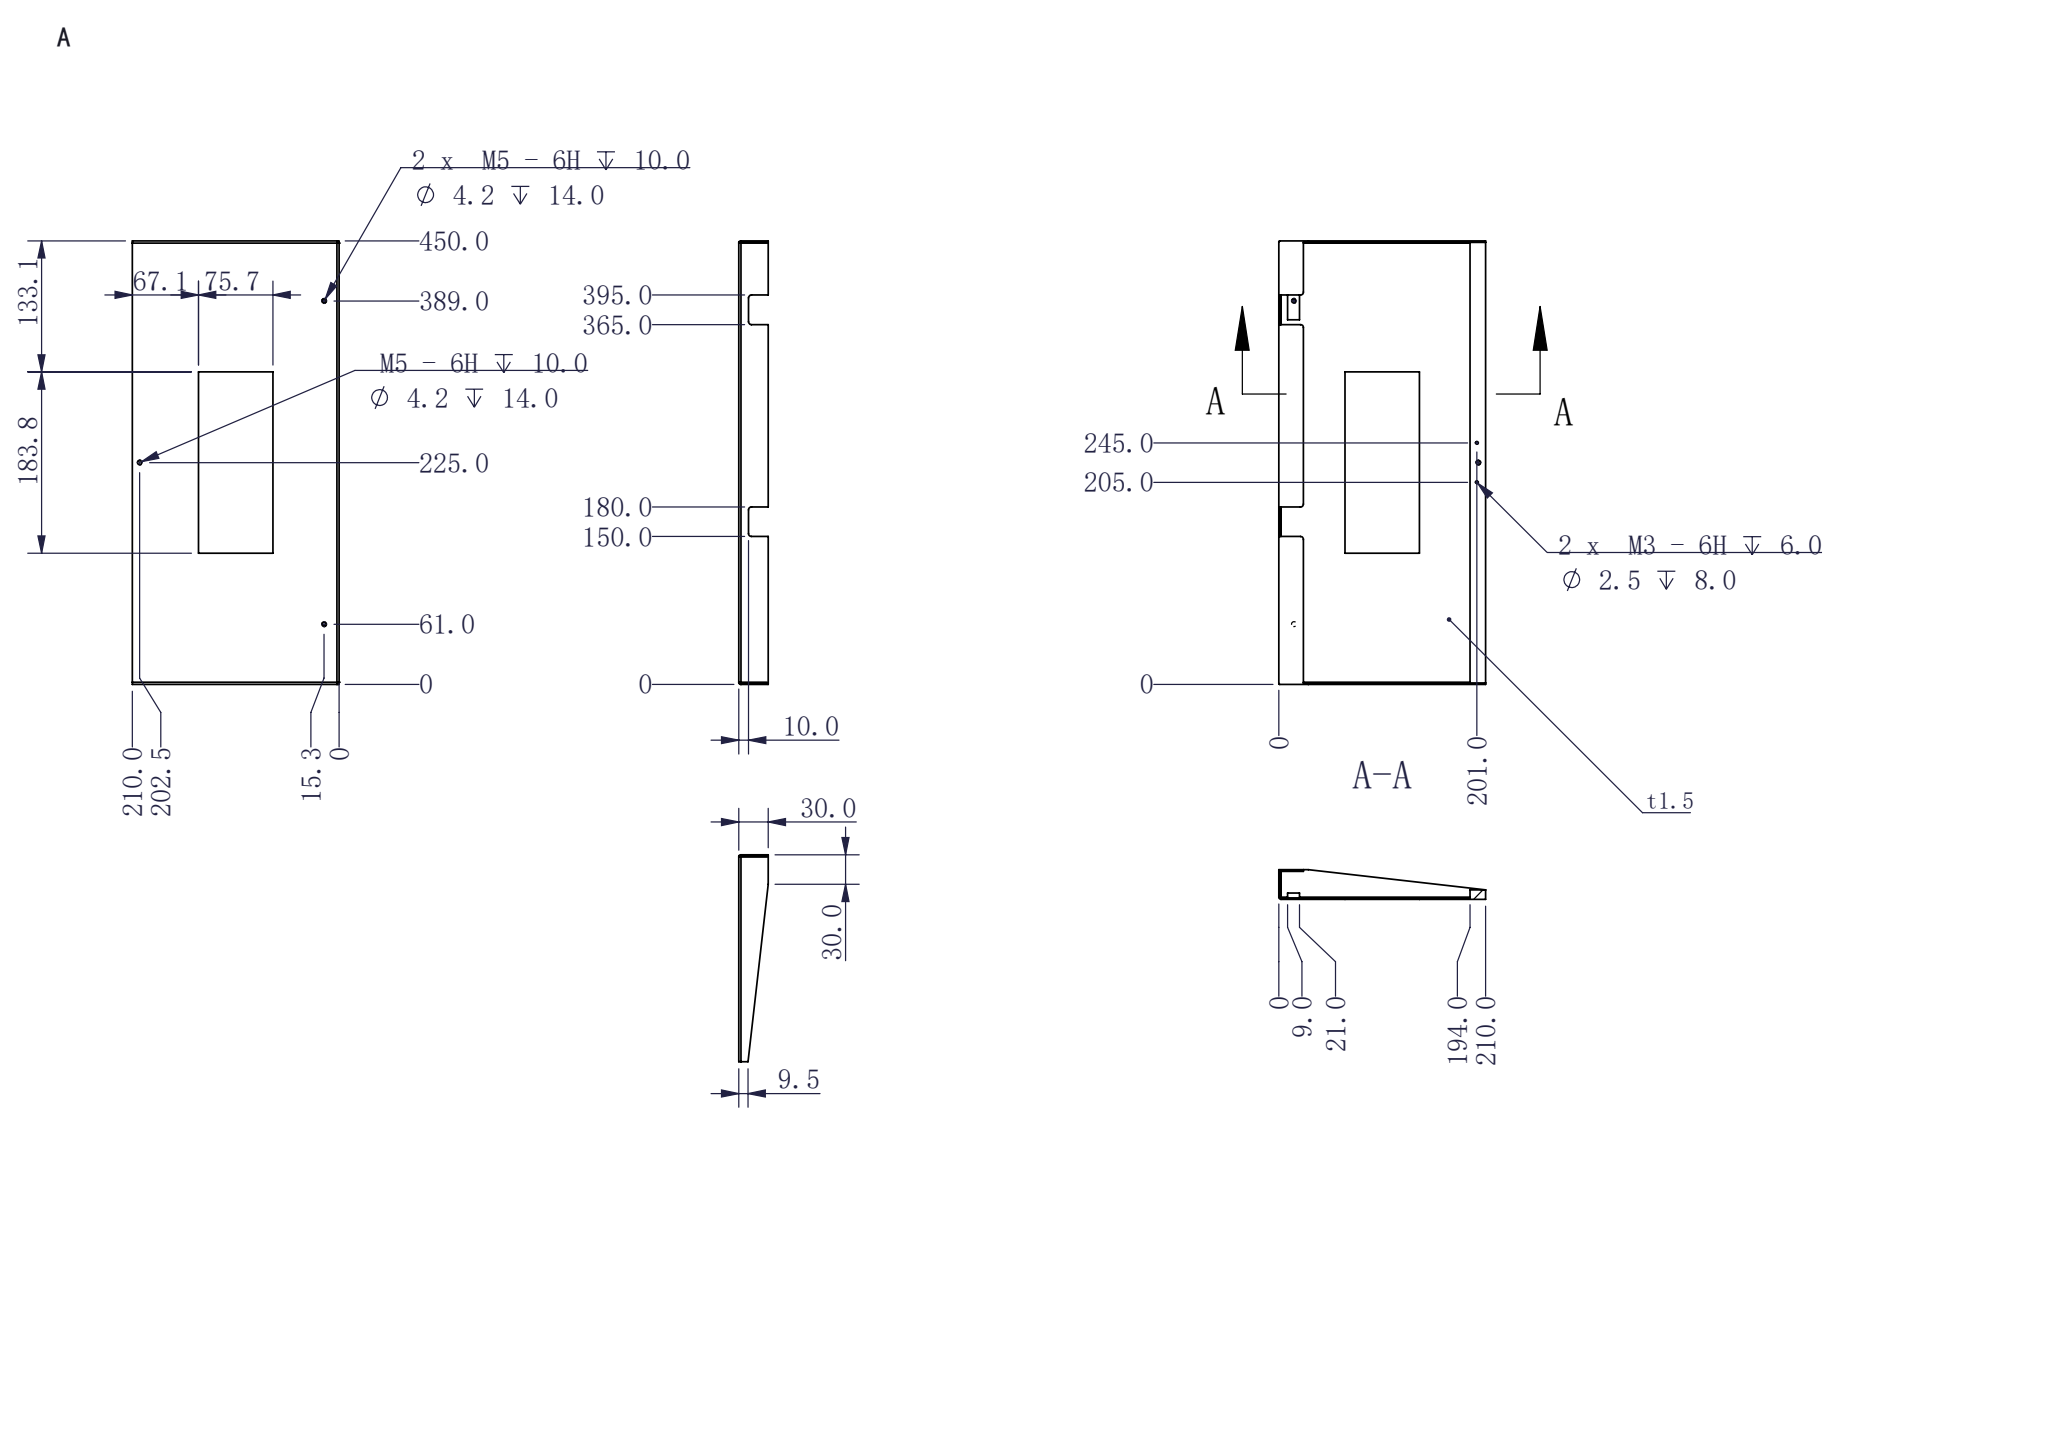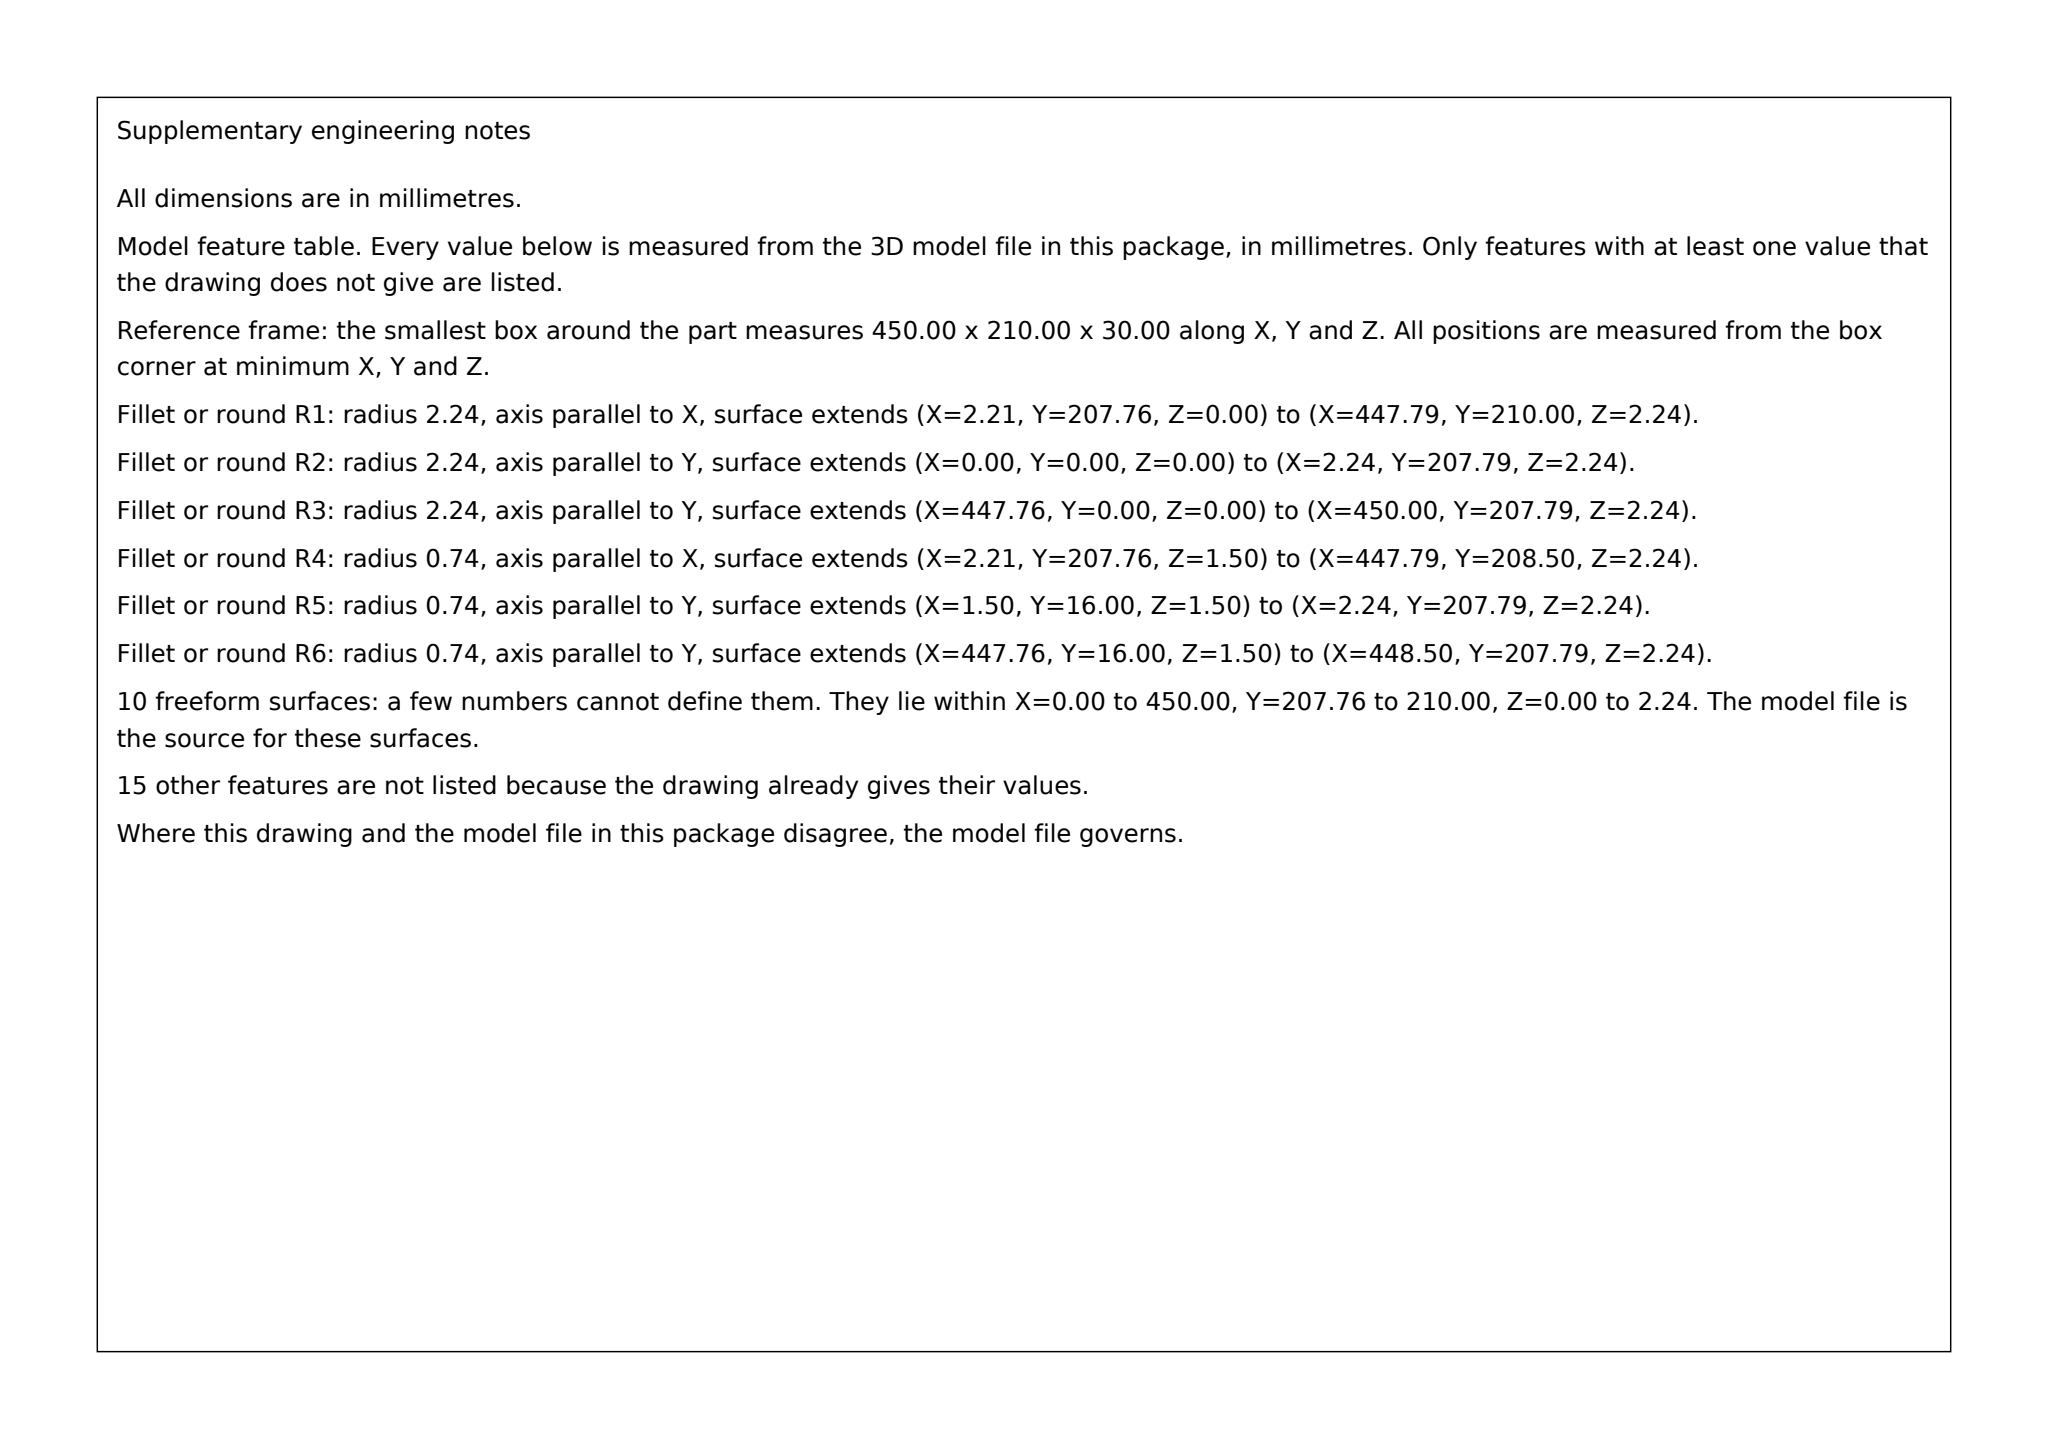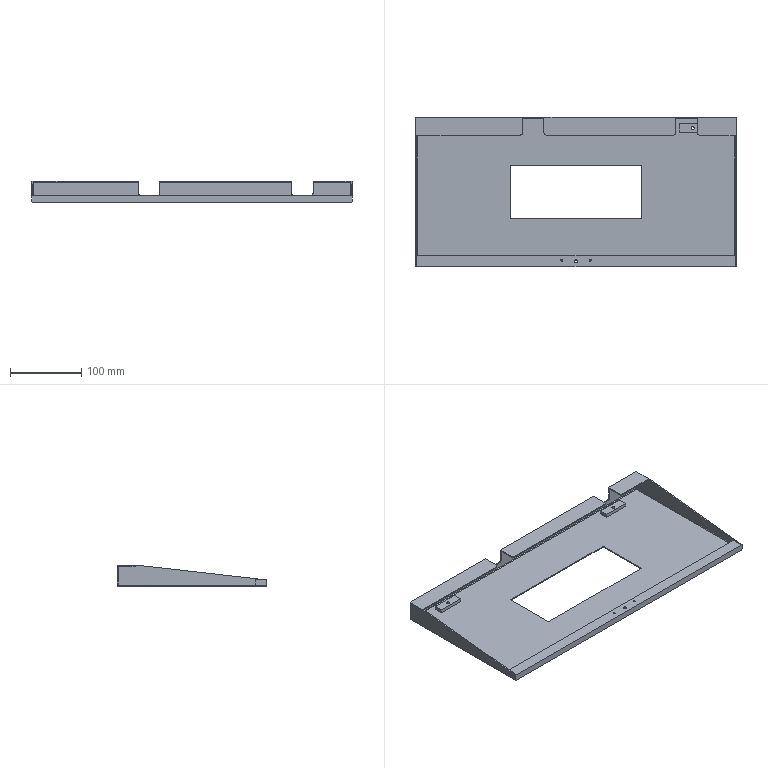Part | SolidWorks | mm | 1 solid | 86 faces | box 450 x 210 x 30 mm | volume 224769 mm3 | plane 46 | cylinder 26 | spline 10 | cone 4 | commonest cylinder face diameters 6 x8 4.2 x6 2.5 x4 1.473 x3 4.473 x3 2 x2
Drawing notes:
ALL BENDS R0.74 INSIDE, R2.24 OUTSIDE, t1.5 | from the solid: Bend cyls dia 1.473 (R0.737) & 4.473 (R2.237) at y207.76, x2.24, x447.76, z2.24
R3 (Ø6) CORNER RELIEF ALL FLANGE NOTCH CORNERS, 8 PL | from the solid: Ø6 cyls: z-axis at x147/183/362/398 (y188); y-axis at x153/177/368/392 (z13) - notches 150-180 & 365-395
2 x Ø2.0 DP 27.8 BEND CORNER RELIEF AT 1.0 & 449.0, 1.0 FR 0 EDGE | from the solid: Ø2.0 z-axis cyls at (1.0,209.0) & (449.0,209.0), L=27.76 from z2.24; drawing y = 210 - y_step = 1.0
A-A: FLANGE NOTCH 38 WIDE, 42.0 TO 80.0, 9.0 DP FR 0 EDGE | from the solid: Planes x=42.0 & x=80.0 (width 38), recess face y_step=201 -> 9.0 from 0 edge
A-A: FLANGE RECESS 38 WIDE, 370.0 TO 408.0, 9.0 DP FR 0 EDGE | from the solid: Planes x=370.0 & x=408.0 (width 38), recess face y_step=201 -> 9.0 from 0 edge
A-A: FLANGE/LIP FACES AT 21.0, 25.0 & 194.0 FR 0 EDGE | from the solid: y planes 189, 185, 16 -> 210-y = 21.0, 25.0, 194.0
M5 HOLE FACES STEPPED TO Z6.5 FR BASE, 2 PL AT 61.0 & 389.0 | from the solid: z plane 6.5 x2; Ø4.2 holes at (61.0,194.7) & (389.0,194.7), L=6.5